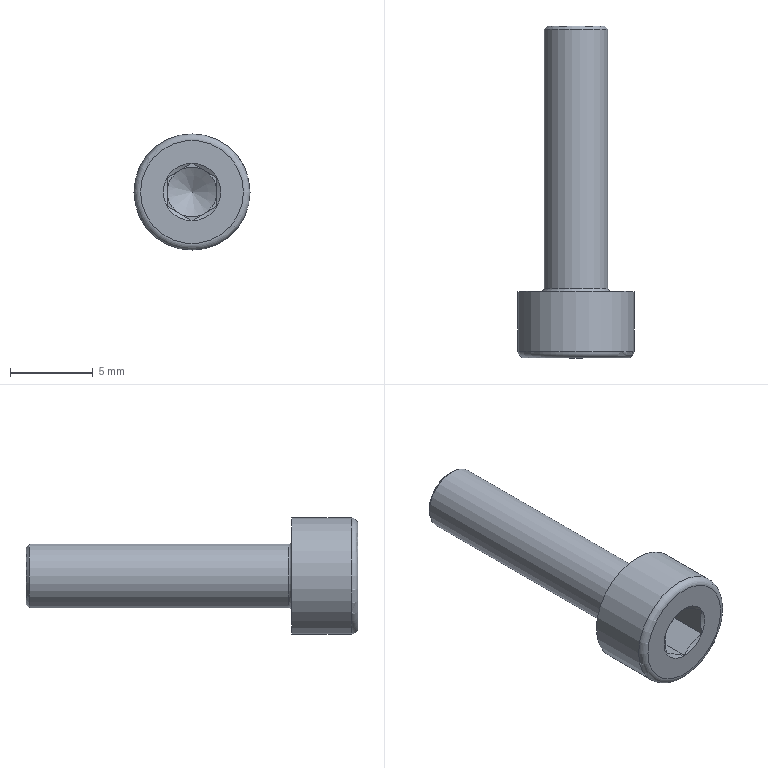Component | NX | GB-T70_1-2000_M4X16 | 1 solid | 27 faces | volume 316 mm3 | plane 15 | cone 8 | cylinder 2 | torus 2 | commonest cylinder face diameters 3.838 x1 7 x1